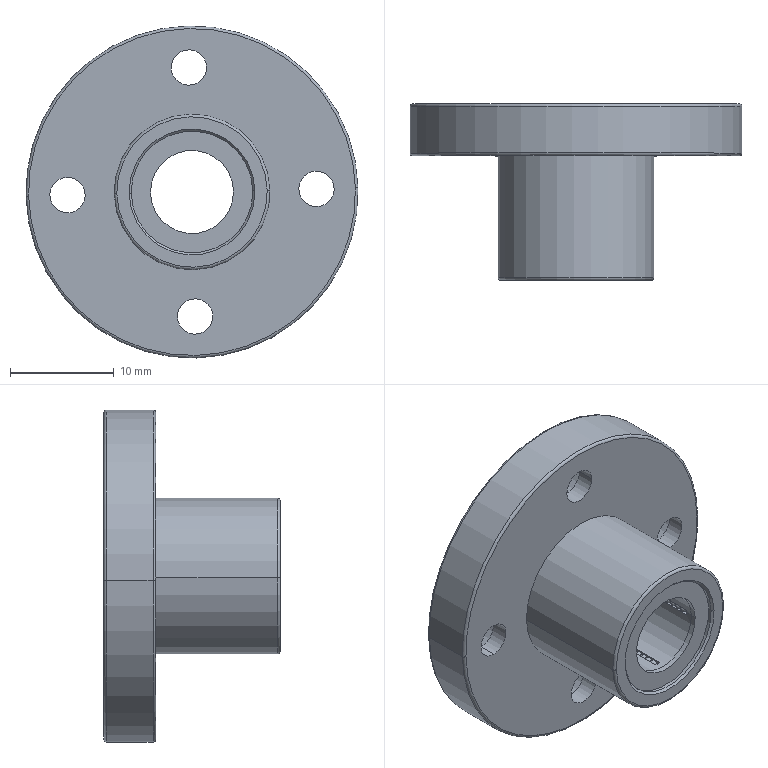Component | SolidWorks | RoundFlangeLinearBearingD8-2 | 3 solids | 568 faces | box 32 x 17 x 32 mm | volume 4719 mm3 | plane 237 | spline 166 | cylinder 79 | sphere 76 | torus 6 | cone 4 | commonest cylinder face diameters 14.98 x28 15 x15 13.25 x8 3.4 x8 6.5 x8 8 x6 11.73 x4 32 x2